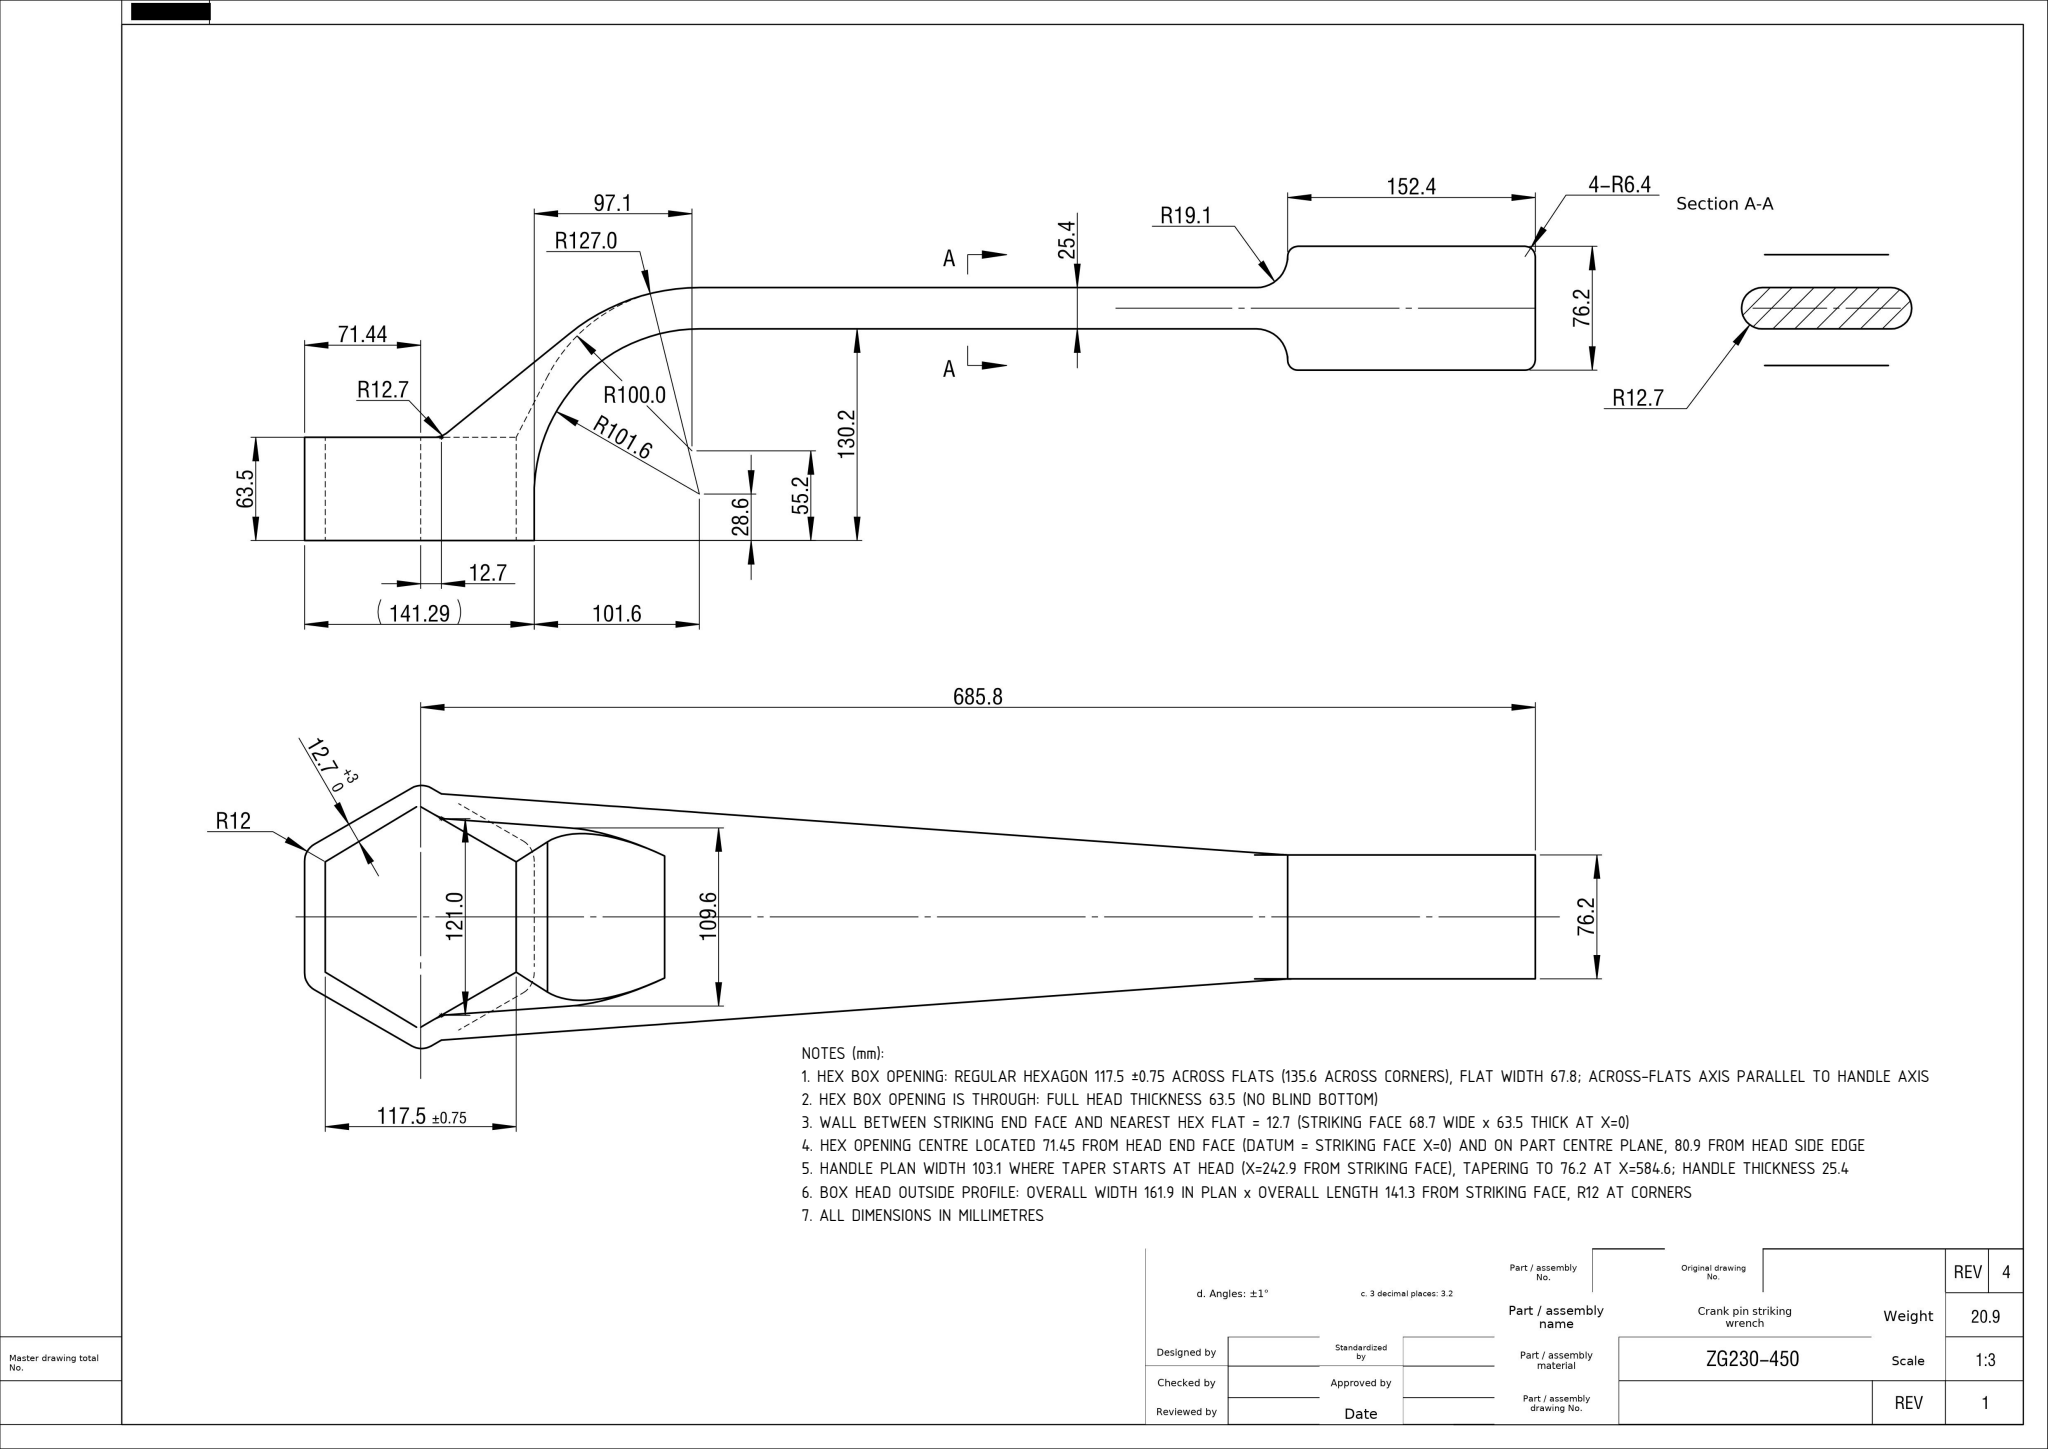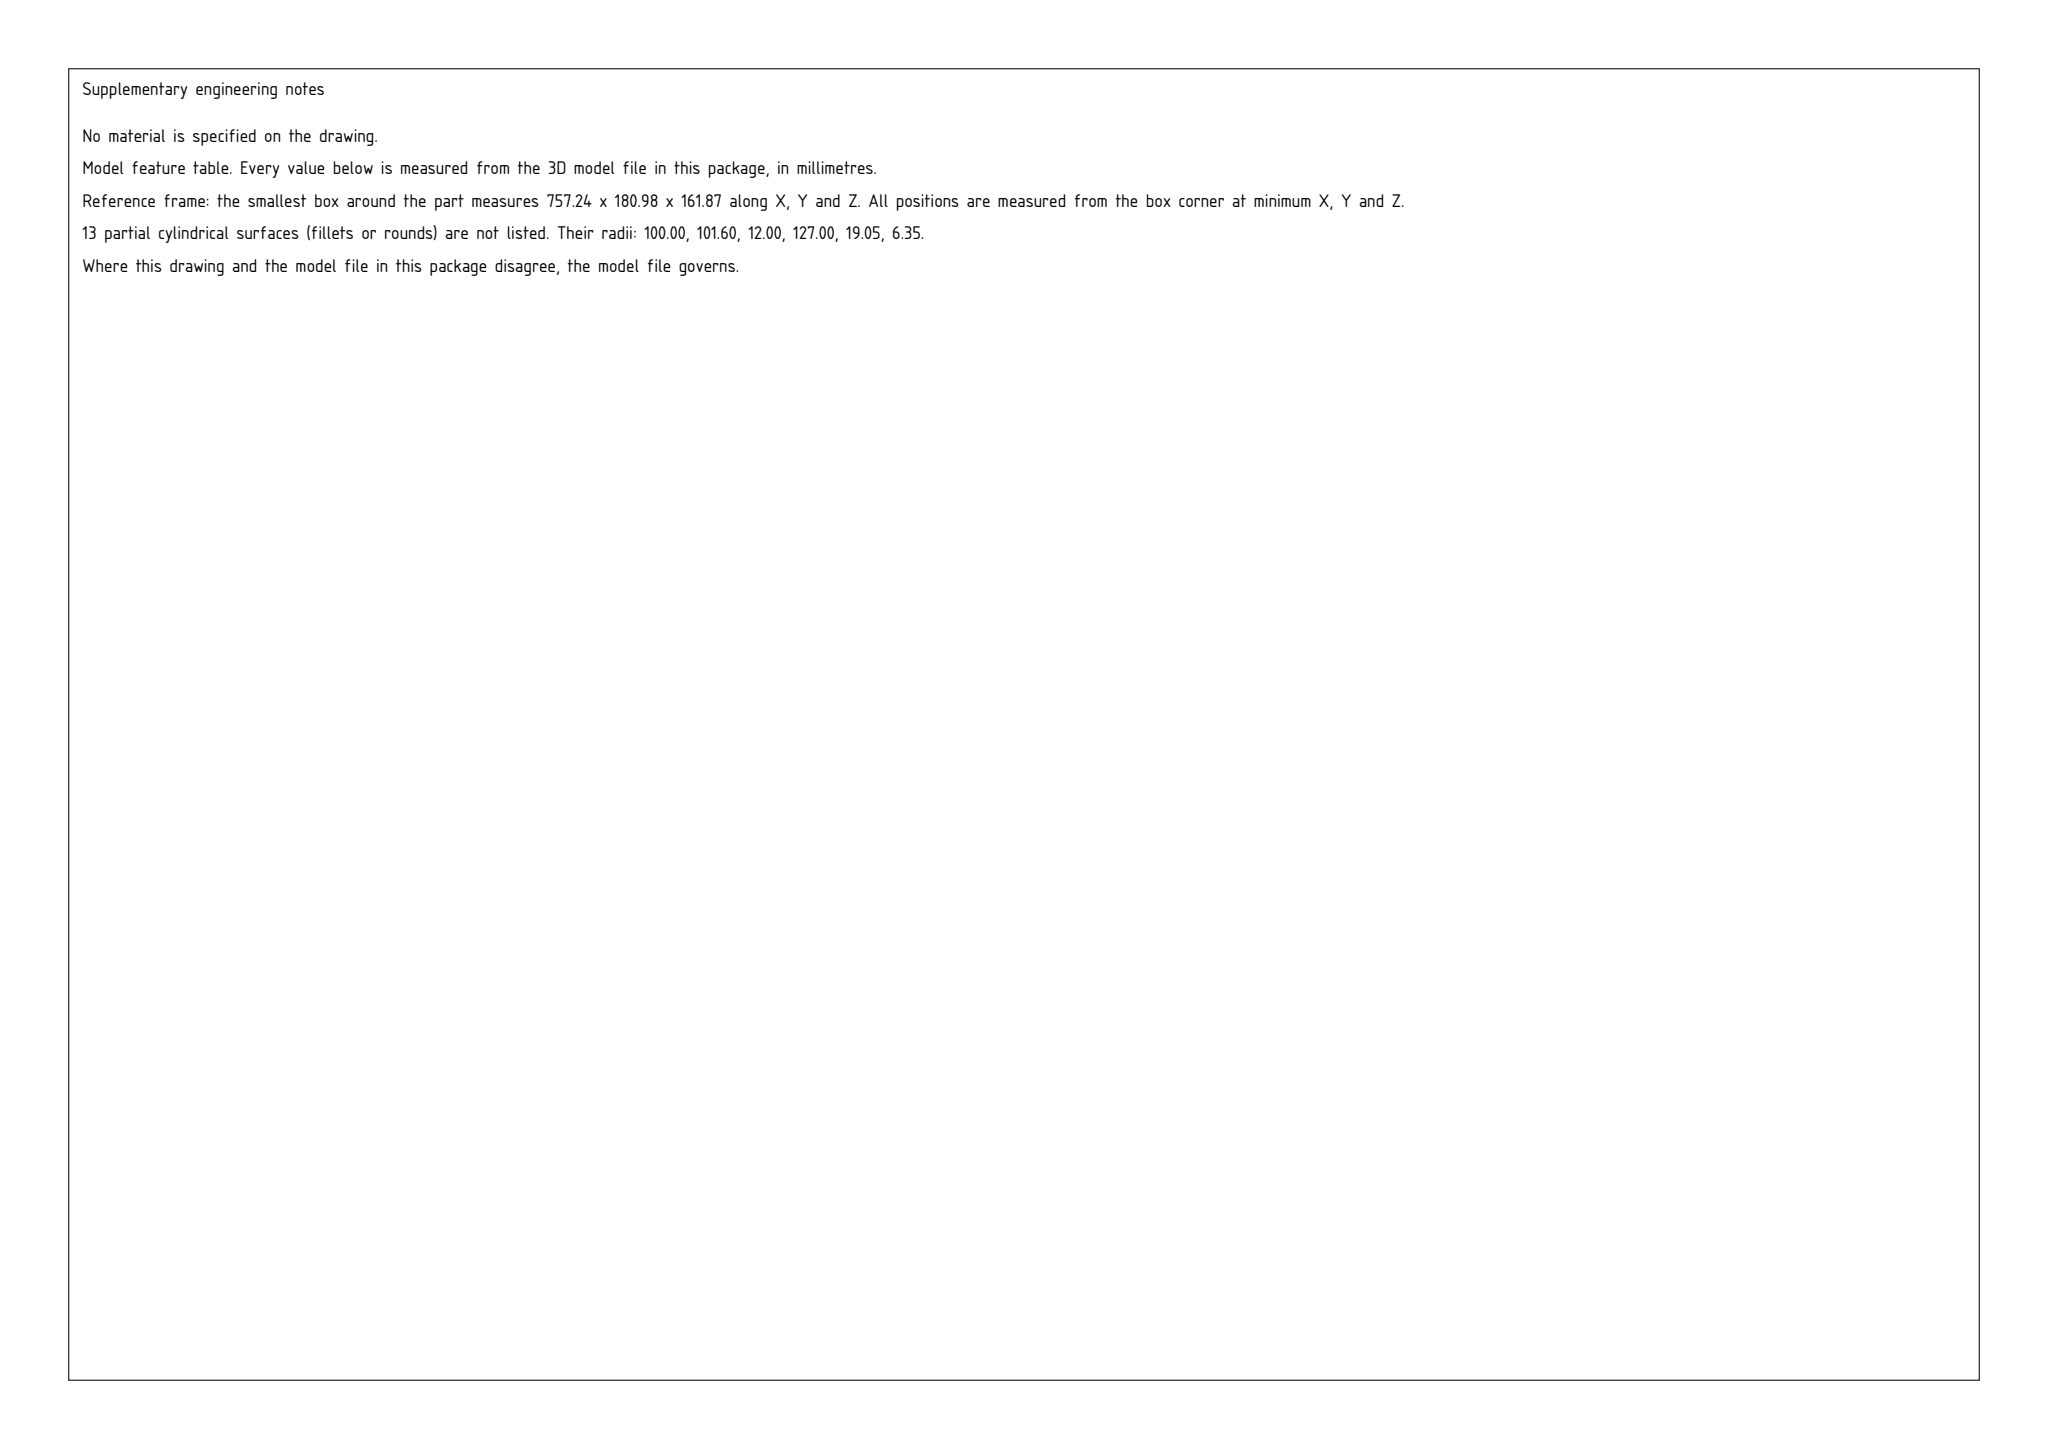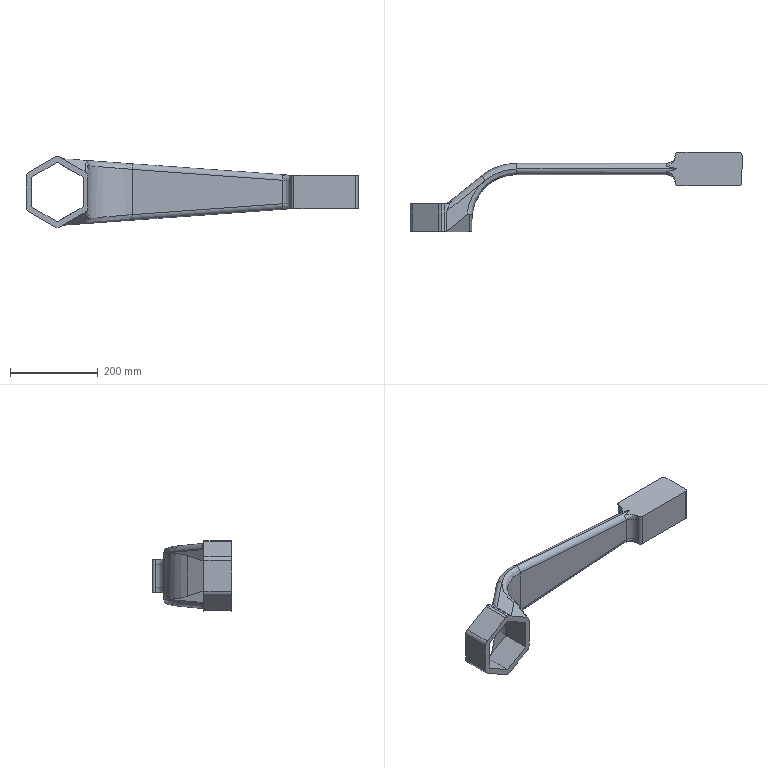Part | SolidWorks | mm | 1 solid | 73 faces | box 757.24 x 180.98 x 161.87 mm | volume 2680701 mm3 | plane 34 | cylinder 22 | spline 13 | torus 4 | commonest cylinder face diameters 24 x7 25.4 x6 12.7 x4 38.1 x2 203.2 x1 254 x1 200 x1
Drawing notes:
HEX BOX OPENING: REGULAR HEXAGON 117.5 ±0.75 ACROSS FLATS (135.6 ACROSS CORNERS), FLAT WIDTH 67.8; ACROSS-FLATS AXIS PARALLEL TO HANDLE AXIS | from the solid: axis_planes x=12.7 and x=130.2, each extent z 47.0-114.8 (two parallel flats 117.5 apart, flat width 67.8); inclined_planes [60,90,30] spanning z 13.1-148.7 (= 135.6 across corners)
HEX BOX OPENING IS THROUGH: FULL HEAD THICKNESS 63.5 (NO BLIND BOTTOM) | from the solid: inclined_planes [60,90,30] bbox_from y=5.6 with size y=63.5, i.e. y 5.6 to 69.1, same as head faces y=5.6 and y=69.1
WALL BETWEEN STRIKING END FACE AND NEAREST HEX FLAT = 12.7 (STRIKING FACE 68.7 WIDE x 63.5 THICK AT X=0) | from the solid: axis_planes x=0.0 extent z 46.6-115.3 area 4358 (end face) and x=12.7 extent z 47.0-114.8 area 4307 (hex flat)
HEX OPENING CENTRE LOCATED 71.45 FROM HEAD END FACE (DATUM = STRIKING FACE X=0) AND ON PART CENTRE PLANE, 80.9 FROM HEAD SIDE EDGE | from the solid: hex flats at x=12.7 and x=130.2 (midpoint 71.45); hex z extent 13.1-148.7 within bbox z 0-161.869 (midpoint 80.9)
HANDLE PLAN WIDTH 103.1 WHERE TAPER STARTS AT HEAD (X=242.9 FROM STRIKING FACE), TAPERING TO 76.2 AT X=584.6; HANDLE THICKNESS 25.4 | from the solid: axis_planes y=135.8 and y=161.2 (25.4 apart) extent x 242.9-585.8, z 29.4-132.5 (=103.1); axis_planes z=42.8 and z=119.0 extent x 584.6-757.2 (=76.2)
BOX HEAD OUTSIDE PROFILE: OVERALL WIDTH 161.9 IN PLAN x OVERALL LENGTH 141.3 FROM STRIKING FACE, R12 AT CORNERS | from the solid: bbox_xyz z = 161.869 and head end faces x=0.0 to x=141.3; cylinders convex arc dia 24.0 axis y at (12.0,115.3), (12.0,46.6), (72.0,12.0), (72.0,149.9)
ALL DIMENSIONS IN MILLIMETRES | from the solid: STEP model facts stated in mm (bbox_xyz 757.239 x 186.624 x 161.869 mm)